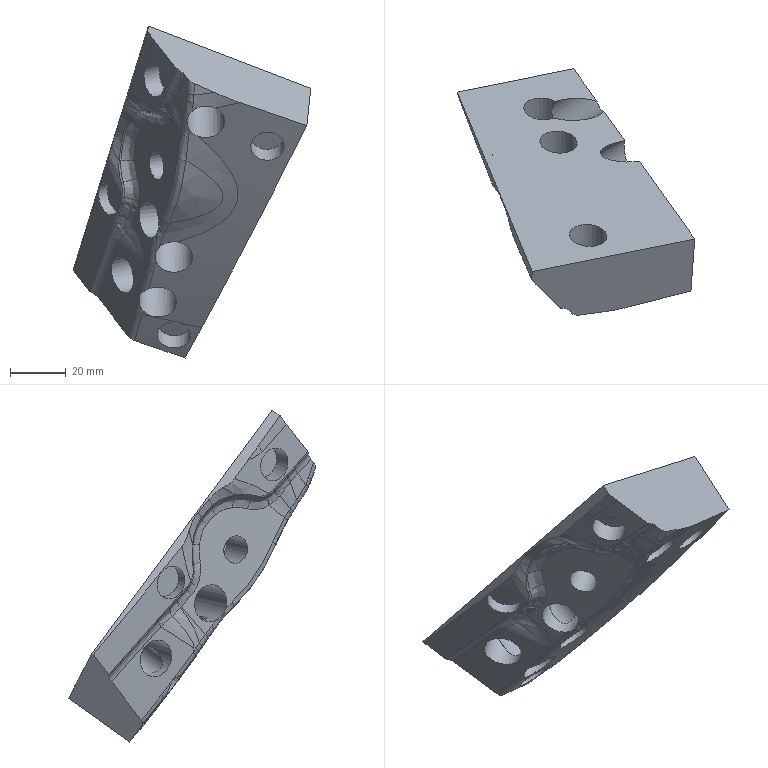CAM job | NX | mm | 3+2-indexed | 1 set-up | 10 operations | part box 85.45 x 88.85 x 119.47
set-up 1
1. Variable-axis Surface Contouring | Mill Mill5 D8 | VARIABLE_CONTOUR | path 214.575 mm | 0.8418 min
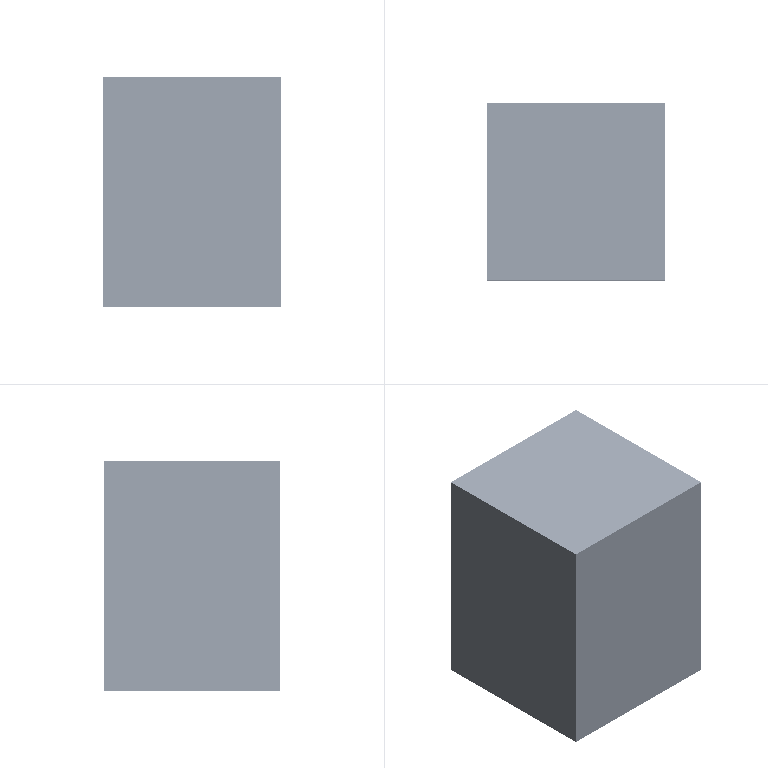2. Variable-axis Surface Contouring | Mill Mill5 D8 | VARIABLE_CONTOUR_COPY | path 1015.563 mm | 4.054 min
3. Variable-axis Surface Contouring | Mill Mill5 D8 | VARIABLE_CONTOUR_COPY_1 | path 893.053 mm | 3.562 min
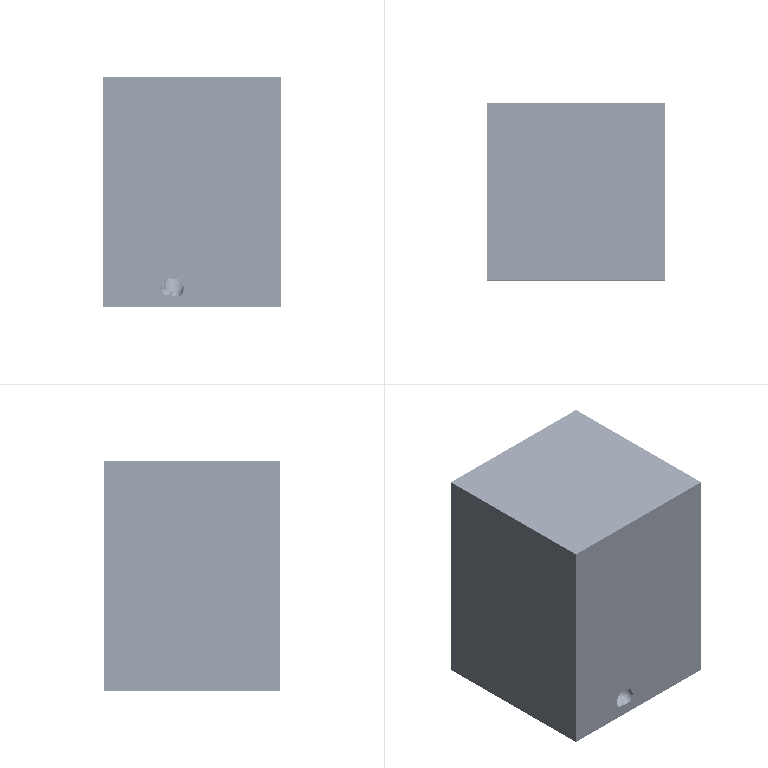4. Variable-axis Surface Contouring | Mill Mill5 D8 | VARIABLE_CONTOUR_COPY_2 | path 219.773 mm | 0.8408 min
5. Variable-axis Surface Contouring | Mill Mill5 D8 | VARIABLE_CONTOUR_COPY_3 | path 898.758 mm | 3.567 min
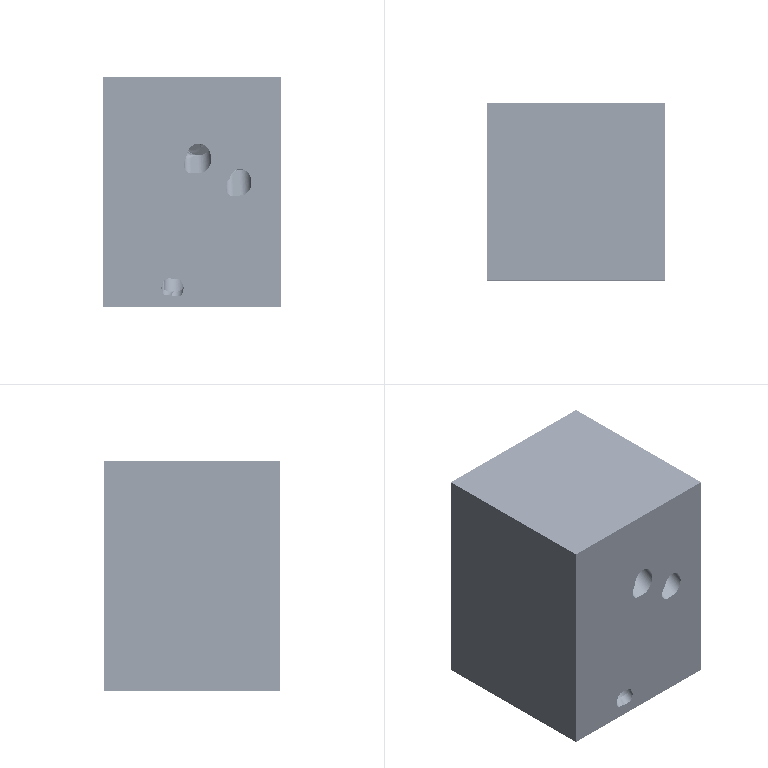6. Variable-axis Surface Contouring | Mill Mill5 D8 | VARIABLE_CONTOUR_COPY_4 | path 242.55 mm | 0.8424 min
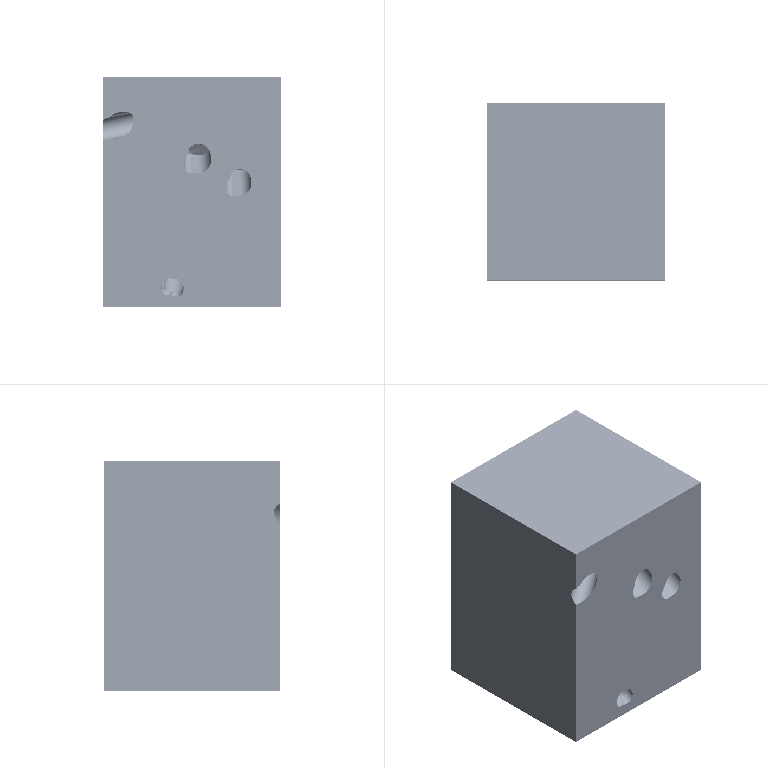7. Variable-axis Surface Contouring | Mill Mill5 D8 | VARIABLE_CONTOUR_COPY_5 | path 349.84 mm | 1.198 min
8. Variable-axis Surface Contouring | Mill Mill5 D8 | VARIABLE_CONTOUR_COPY_6 | path 1109.842 mm | 4.26 min
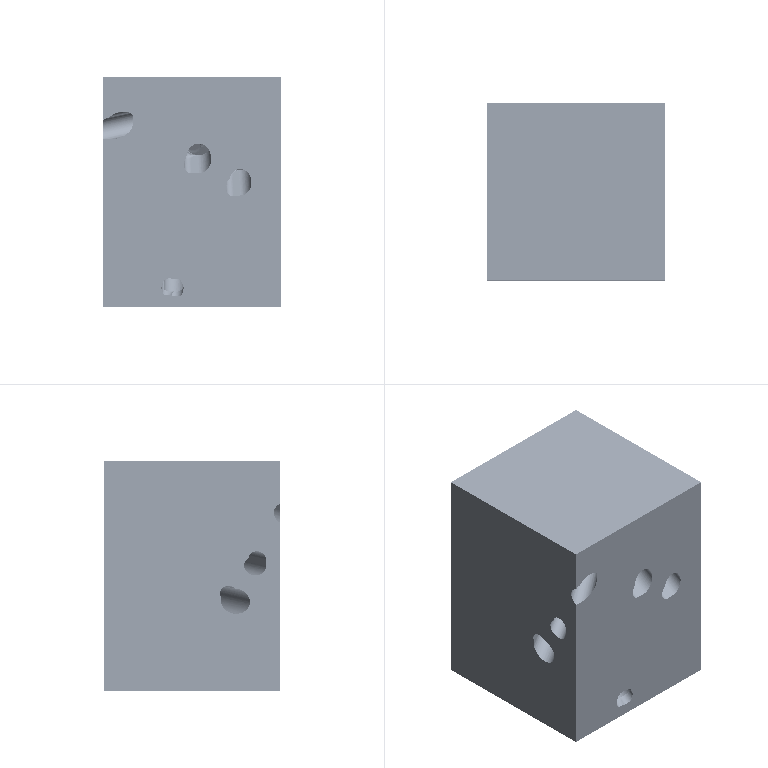9. Variable-axis Surface Contouring | Mill Mill5 D8 | VARIABLE_CONTOUR_COPY_7 | path 260.21 mm | 0.8438 min
10. Variable-axis Surface Contouring | Mill Mill5 D8 | VARIABLE_CONTOUR_COPY_8 | path 939.831 mm | 3.566 min